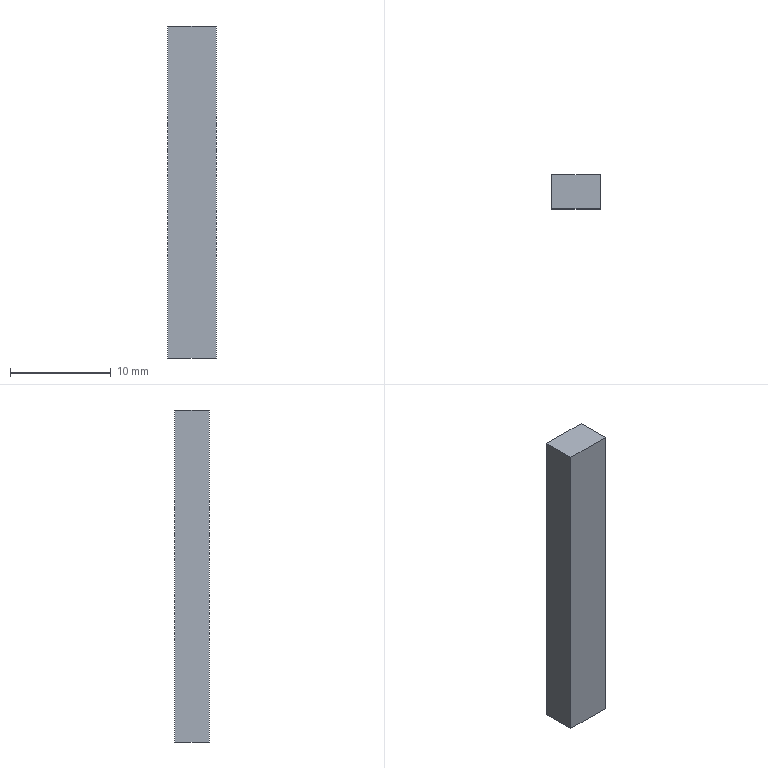Component | SolidWorks | MiddleShortPlate-1 | 1 solid | 6 faces | box 4.85 x 3.4 x 33 mm | volume 544 mm3 | plane 6
build123d program:
from build123d import *

# Parameters (mm, degrees)
SKETCH1_W           = 4.845
SKETCH1_H           = 3.401
BOSS_EXTRUDE1_DEPTH = 33


with BuildPart() as part:
    # Sketch1 → Boss-Extrude1 (new body)
    with BuildSketch(Plane.XY):
        with Locations((-131.102, -23.125)):
            Rectangle(SKETCH1_W, SKETCH1_H)
    extrude(amount=BOSS_EXTRUDE1_DEPTH)


solid = part.part

# Placed as in the assembly
solid = solid.moved(Location((247.958, 0.05541, -15.5), (0, 0, 0)))
STEP:
#1=COLOUR_RGB('',0.7922,0.8196,0.9333);
#2=FILL_AREA_STYLE_COLOUR('',#1);
#3=FILL_AREA_STYLE('',(#2));
#4=SURFACE_STYLE_FILL_AREA(#3);
#5=SURFACE_SIDE_STYLE('',(#4));
#6=SURFACE_STYLE_USAGE(.BOTH.,#5);
#7=PRESENTATION_STYLE_ASSIGNMENT((#6));
#8=CARTESIAN_POINT('',(4.696,-0.8413,0.689));
#9=VERTEX_POINT('',#8);
#10=CARTESIAN_POINT('',(4.696,-0.9752,0.689));
#11=VERTEX_POINT('',#10);
#12=CARTESIAN_POINT('',(4.696,-0.8413,0.689));
#13=DIRECTION('',(0.,-1.,0.));
#14=VECTOR('',#13,39.37);
#15=LINE('',#12,#14);
#16=EDGE_CURVE('',#9,#11,#15,.T.);
#17=ORIENTED_EDGE('',*,*,#16,.T.);
#18=CARTESIAN_POINT('',(4.696,-0.9752,-0.6102));
#19=VERTEX_POINT('',#18);
#20=CARTESIAN_POINT('',(4.696,-0.9752,-0.6102));
#21=DIRECTION('',(0.,0.,1.));
#22=VECTOR('',#21,39.37);
#23=LINE('',#20,#22);
#24=EDGE_CURVE('',#19,#11,#23,.T.);
#25=ORIENTED_EDGE('',*,*,#24,.F.);
#26=CARTESIAN_POINT('',(4.696,-0.8413,-0.6102));
#27=VERTEX_POINT('',#26);
#28=CARTESIAN_POINT('',(4.696,-0.8413,-0.6102));
#29=DIRECTION('',(0.,-1.,0.));
#30=VECTOR('',#29,39.37);
#31=LINE('',#28,#30);
#32=EDGE_CURVE('',#27,#19,#31,.T.);
#33=ORIENTED_EDGE('',*,*,#32,.F.);
#34=CARTESIAN_POINT('',(4.696,-0.8413,-0.6102));
#35=DIRECTION('',(0.,0.,1.));
#36=VECTOR('',#35,39.37);
#37=LINE('',#34,#36);
#38=EDGE_CURVE('',#27,#9,#37,.T.);
#39=ORIENTED_EDGE('',*,*,#38,.T.);
#40=EDGE_LOOP('',(#17,#25,#33,#39));
#41=FACE_OUTER_BOUND('',#40,.T.);
#42=CARTESIAN_POINT('',(4.696,-0.8413,-0.6102));
#43=DIRECTION('',(-1.,0.,0.));
#44=DIRECTION('',(0.,0.,1.));
#45=AXIS2_PLACEMENT_3D('',#42,#43,#44);
#46=PLANE('',#45);
#47=ADVANCED_FACE('',(#41),#46,.F.);
#48=CARTESIAN_POINT('',(4.505,-0.9752,0.689));
#49=VERTEX_POINT('',#48);
#50=CARTESIAN_POINT('',(4.696,-0.9752,0.689));
#51=DIRECTION('',(-1.,0.,0.));
#52=VECTOR('',#51,39.37);
#53=LINE('',#50,#52);
#54=EDGE_CURVE('',#11,#49,#53,.T.);
#55=ORIENTED_EDGE('',*,*,#54,.T.);
#56=CARTESIAN_POINT('',(4.505,-0.9752,-0.6102));
#57=VERTEX_POINT('',#56);
#58=CARTESIAN_POINT('',(4.505,-0.9752,-0.6102));
#59=DIRECTION('',(0.,0.,1.));
#60=VECTOR('',#59,39.37);
#61=LINE('',#58,#60);
#62=EDGE_CURVE('',#57,#49,#61,.T.);
#63=ORIENTED_EDGE('',*,*,#62,.F.);
#64=CARTESIAN_POINT('',(4.696,-0.9752,-0.6102));
#65=DIRECTION('',(-1.,0.,0.));
#66=VECTOR('',#65,39.37);
#67=LINE('',#64,#66);
#68=EDGE_CURVE('',#19,#57,#67,.T.);
#69=ORIENTED_EDGE('',*,*,#68,.F.);
#70=ORIENTED_EDGE('',*,*,#24,.T.);
#71=EDGE_LOOP('',(#55,#63,#69,#70));
#72=FACE_OUTER_BOUND('',#71,.T.);
#73=CARTESIAN_POINT('',(4.696,-0.9752,-0.6102));
#74=DIRECTION('',(0.,1.,0.));
#75=DIRECTION('',(0.,0.,-1.));
#76=AXIS2_PLACEMENT_3D('',#73,#74,#75);
#77=PLANE('',#76);
#78=ADVANCED_FACE('',(#72),#77,.F.);
#79=CARTESIAN_POINT('',(4.505,-0.8413,0.689));
#80=VERTEX_POINT('',#79);
#81=CARTESIAN_POINT('',(4.505,-0.8413,0.689));
#82=DIRECTION('',(0.,1.,0.));
#83=VECTOR('',#82,39.37);
#84=LINE('',#81,#83);
#85=EDGE_CURVE('',#49,#80,#84,.T.);
#86=ORIENTED_EDGE('',*,*,#85,.T.);
#87=CARTESIAN_POINT('',(4.505,-0.8413,-0.6102));
#88=VERTEX_POINT('',#87);
#89=CARTESIAN_POINT('',(4.505,-0.8413,-0.6102));
#90=DIRECTION('',(0.,0.,1.));
#91=VECTOR('',#90,39.37);
#92=LINE('',#89,#91);
#93=EDGE_CURVE('',#88,#80,#92,.T.);
#94=ORIENTED_EDGE('',*,*,#93,.F.);
#95=CARTESIAN_POINT('',(4.505,-0.8413,-0.6102));
#96=DIRECTION('',(0.,1.,0.));
#97=VECTOR('',#96,39.37);
#98=LINE('',#95,#97);
#99=EDGE_CURVE('',#57,#88,#98,.T.);
#100=ORIENTED_EDGE('',*,*,#99,.F.);
#101=ORIENTED_EDGE('',*,*,#62,.T.);
#102=EDGE_LOOP('',(#86,#94,#100,#101));
#103=FACE_OUTER_BOUND('',#102,.T.);
#104=CARTESIAN_POINT('',(4.505,-0.8413,-0.6102));
#105=DIRECTION('',(1.,0.,0.));
#106=DIRECTION('',(0.,0.,-1.));
#107=AXIS2_PLACEMENT_3D('',#104,#105,#106);
#108=PLANE('',#107);
#109=ADVANCED_FACE('',(#103),#108,.F.);
#110=CARTESIAN_POINT('',(4.696,-0.8413,0.689));
#111=DIRECTION('',(1.,0.,0.));
#112=VECTOR('',#111,39.37);
#113=LINE('',#110,#112);
#114=EDGE_CURVE('',#80,#9,#113,.T.);
#115=ORIENTED_EDGE('',*,*,#114,.T.);
#116=ORIENTED_EDGE('',*,*,#38,.F.);
#117=CARTESIAN_POINT('',(4.696,-0.8413,-0.6102));
#118=DIRECTION('',(1.,0.,0.));
#119=VECTOR('',#118,39.37);
#120=LINE('',#117,#119);
#121=EDGE_CURVE('',#88,#27,#120,.T.);
#122=ORIENTED_EDGE('',*,*,#121,.F.);
#123=ORIENTED_EDGE('',*,*,#93,.T.);
#124=EDGE_LOOP('',(#115,#116,#122,#123));
#125=FACE_OUTER_BOUND('',#124,.T.);
#126=CARTESIAN_POINT('',(4.696,-0.8413,-0.6102));
#127=DIRECTION('',(0.,-1.,0.));
#128=DIRECTION('',(0.,0.,1.));
#129=AXIS2_PLACEMENT_3D('',#126,#127,#128);
#130=PLANE('',#129);
#131=ADVANCED_FACE('',(#125),#130,.F.);
#132=ORIENTED_EDGE('',*,*,#32,.T.);
#133=ORIENTED_EDGE('',*,*,#68,.T.);
#134=ORIENTED_EDGE('',*,*,#99,.T.);
#135=ORIENTED_EDGE('',*,*,#121,.T.);
#136=EDGE_LOOP('',(#132,#133,#134,#135));
#137=FACE_OUTER_BOUND('',#136,.T.);
#138=CARTESIAN_POINT('',(-0.5609,0.002181,-0.6102));
#139=DIRECTION('',(0.,0.,-1.));
#140=DIRECTION('',(-1.,0.,0.));
#141=AXIS2_PLACEMENT_3D('',#138,#139,#140);
#142=PLANE('',#141);
#143=ADVANCED_FACE('',(#137),#142,.T.);
#144=ORIENTED_EDGE('',*,*,#16,.F.);
#145=ORIENTED_EDGE('',*,*,#114,.F.);
#146=ORIENTED_EDGE('',*,*,#85,.F.);
#147=ORIENTED_EDGE('',*,*,#54,.F.);
#148=EDGE_LOOP('',(#144,#145,#146,#147));
#149=FACE_OUTER_BOUND('',#148,.T.);
#150=CARTESIAN_POINT('',(-0.5609,0.002181,0.689));
#151=DIRECTION('',(0.,0.,-1.));
#152=DIRECTION('',(-1.,0.,0.));
#153=AXIS2_PLACEMENT_3D('',#150,#151,#152);
#154=PLANE('',#153);
#155=ADVANCED_FACE('',(#149),#154,.F.);
#156=CLOSED_SHELL('',(#47,#78,#109,#131,#143,#155));
#157=MANIFOLD_SOLID_BREP('',#156);
#158=STYLED_ITEM('',(#7),#157);
#159=PRESENTATION_LAYER_ASSIGNMENT('','',(#158));
#160=(LENGTH_UNIT()NAMED_UNIT(*)SI_UNIT($,.METRE.));
#161=LENGTH_MEASURE_WITH_UNIT(LENGTH_MEASURE(0.0254),#160);
#162=DIMENSIONAL_EXPONENTS(1.,0.,0.,0.,0.,0.,0.);
#163=(CONVERSION_BASED_UNIT('',#161)LENGTH_UNIT()NAMED_UNIT(#162));
#164=UNCERTAINTY_MEASURE_WITH_UNIT(LENGTH_MEASURE(0.00001),#163,'','');
#165=(NAMED_UNIT(*)PLANE_ANGLE_UNIT()SI_UNIT($,.RADIAN.));
#166=(NAMED_UNIT(*)SI_UNIT($,.STERADIAN.)SOLID_ANGLE_UNIT());
#167=(GEOMETRIC_REPRESENTATION_CONTEXT(3)GLOBAL_UNCERTAINTY_ASSIGNED_CONTEXT((#164))GLOBAL_UNIT_ASSIGNED_CONTEXT((#163,#165,#166))REPRESENTATION_CONTEXT('',''));
#168=MECHANICAL_DESIGN_GEOMETRIC_PRESENTATION_REPRESENTATION('',(#158),#167);
#169=CARTESIAN_POINT('',(0.,0.,0.));
#170=DIRECTION('',(0.,0.,1.));
#171=DIRECTION('',(1.,0.,0.));
#172=AXIS2_PLACEMENT_3D('',#169,#170,#171);
#173=(LENGTH_UNIT()NAMED_UNIT(*)SI_UNIT($,.METRE.));
#174=LENGTH_MEASURE_WITH_UNIT(LENGTH_MEASURE(0.0254),#173);
#175=DIMENSIONAL_EXPONENTS(1.,0.,0.,0.,0.,0.,0.);
#176=(CONVERSION_BASED_UNIT('',#174)LENGTH_UNIT()NAMED_UNIT(#175));
#177=UNCERTAINTY_MEASURE_WITH_UNIT(LENGTH_MEASURE(0.00001),#176,'','');
#178=(NAMED_UNIT(*)PLANE_ANGLE_UNIT()SI_UNIT($,.RADIAN.));
#179=(NAMED_UNIT(*)SI_UNIT($,.STERADIAN.)SOLID_ANGLE_UNIT());
#180=(GEOMETRIC_REPRESENTATION_CONTEXT(3)GLOBAL_UNCERTAINTY_ASSIGNED_CONTEXT((#177))GLOBAL_UNIT_ASSIGNED_CONTEXT((#176,#178,#179))REPRESENTATION_CONTEXT('',''));
#181=ADVANCED_BREP_SHAPE_REPRESENTATION('',(#157,#172),#180);